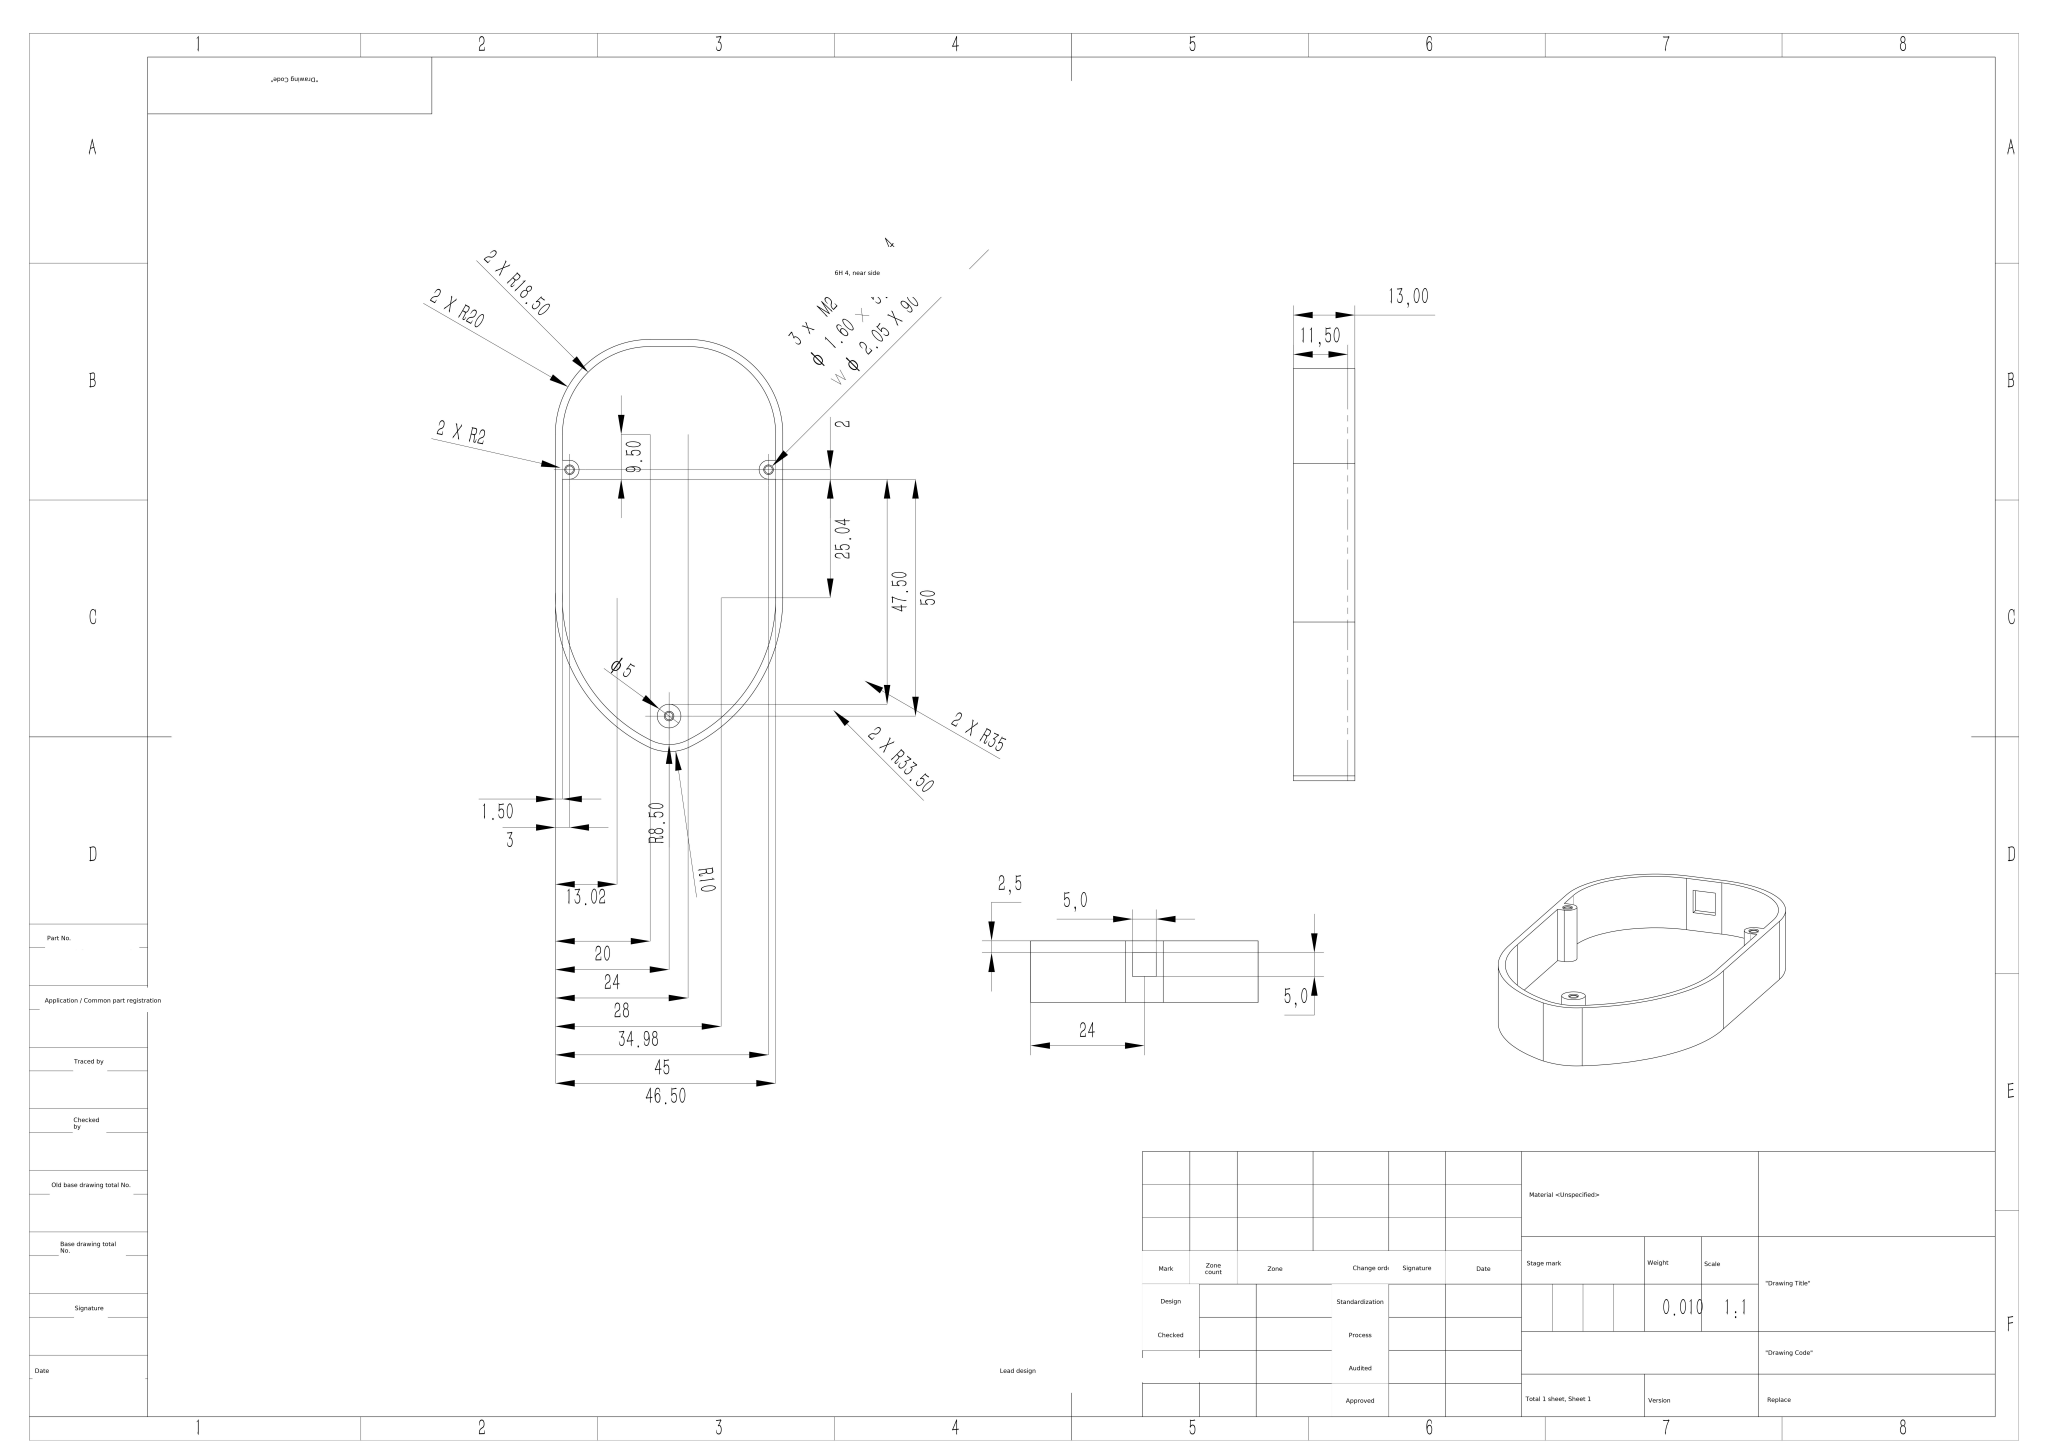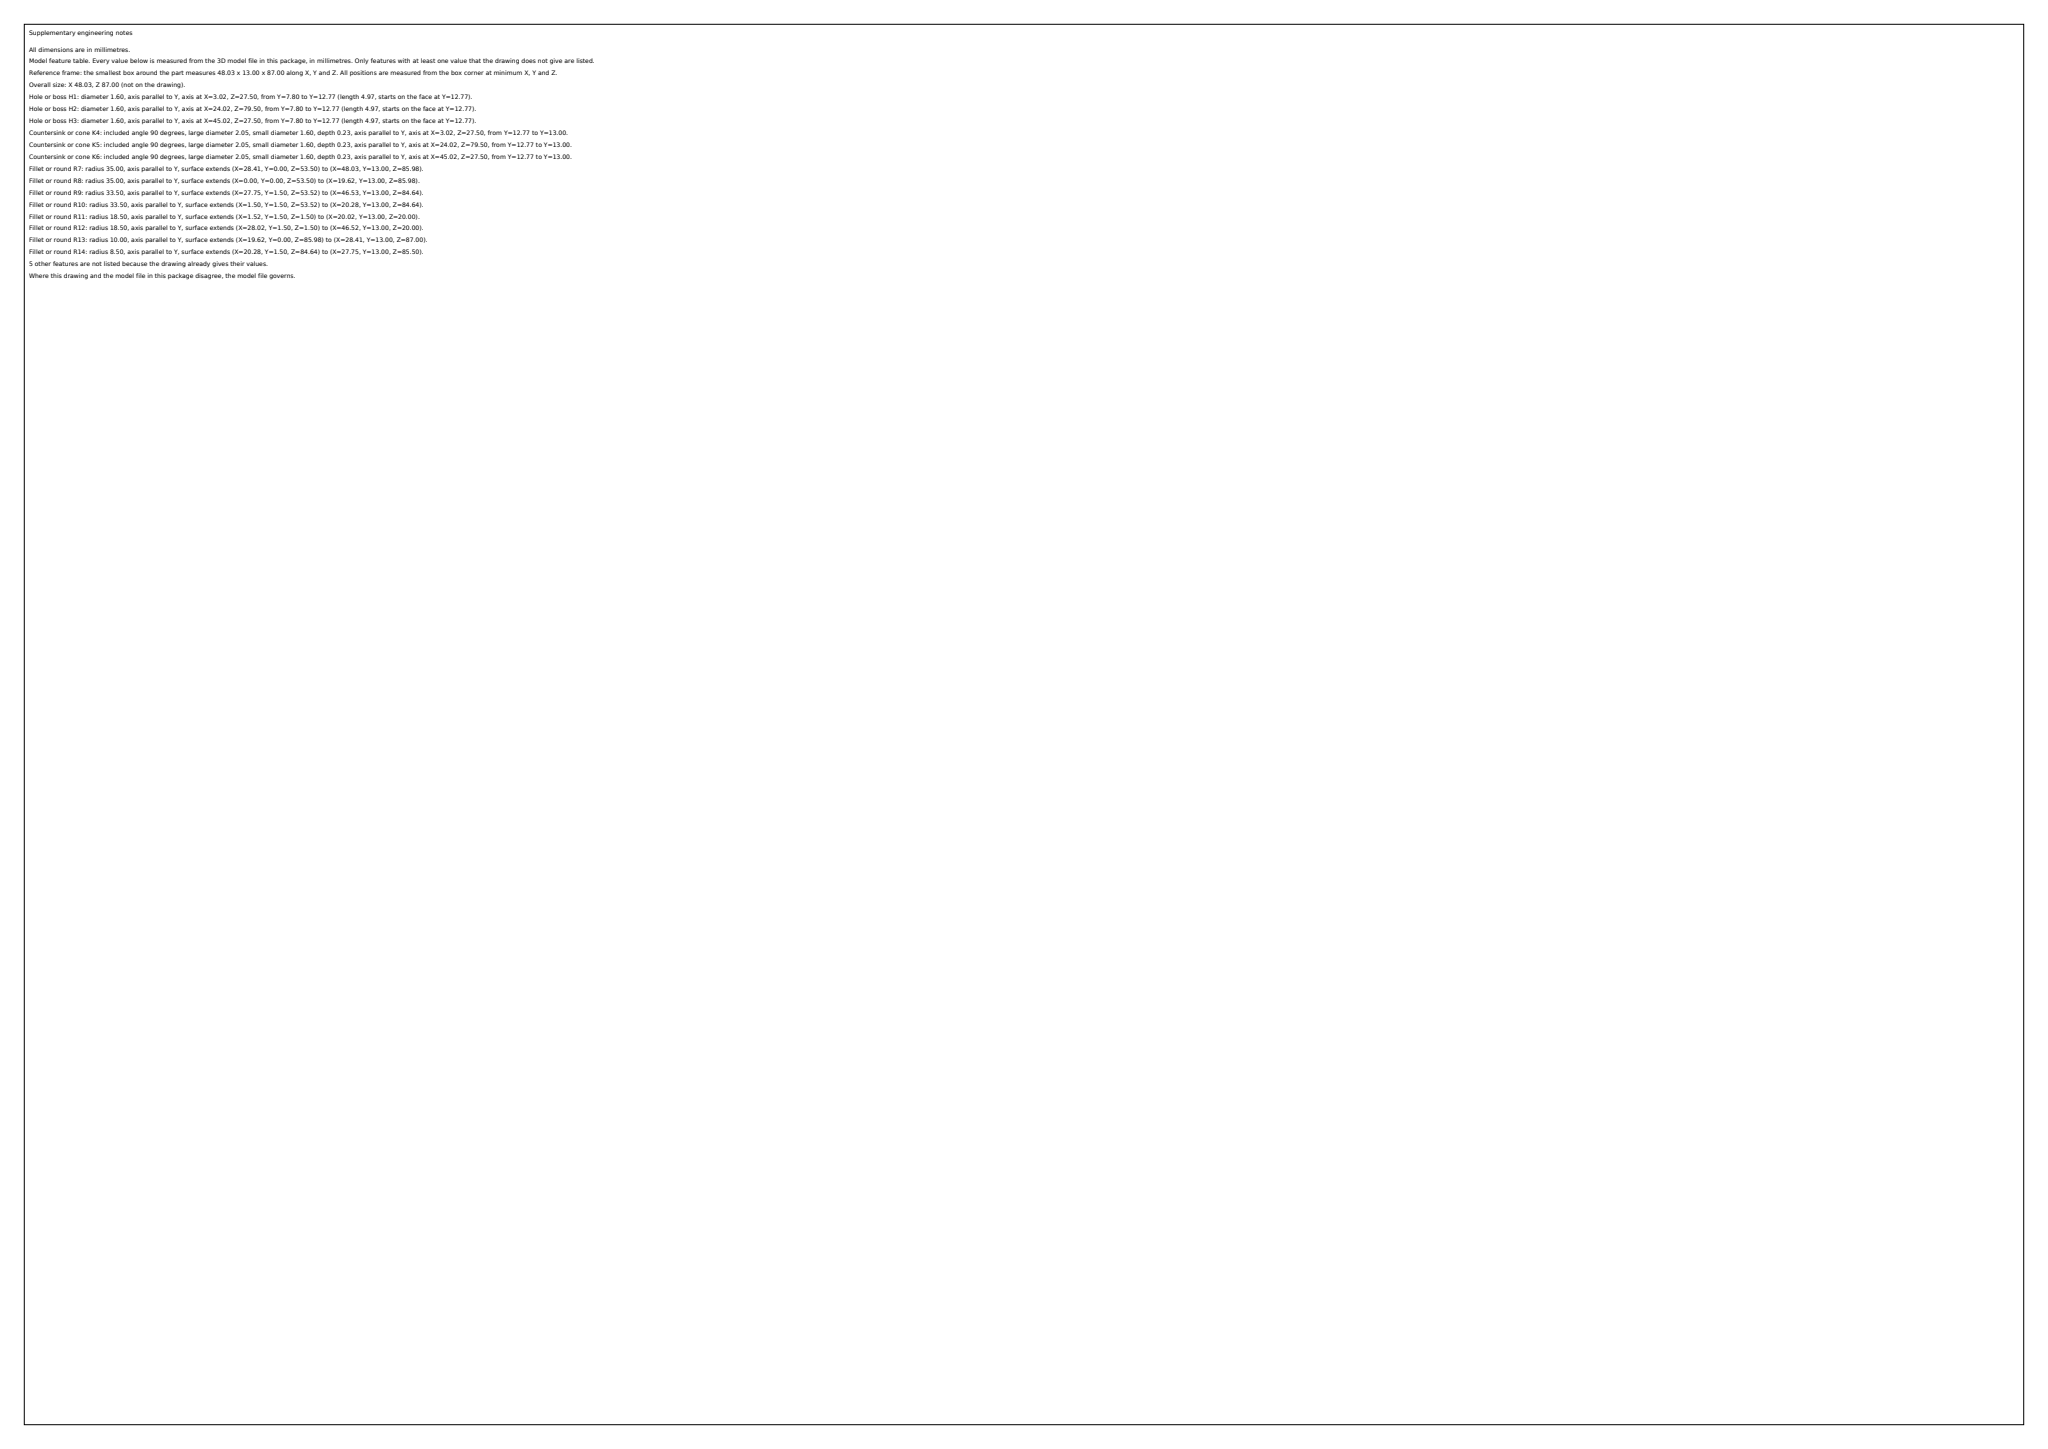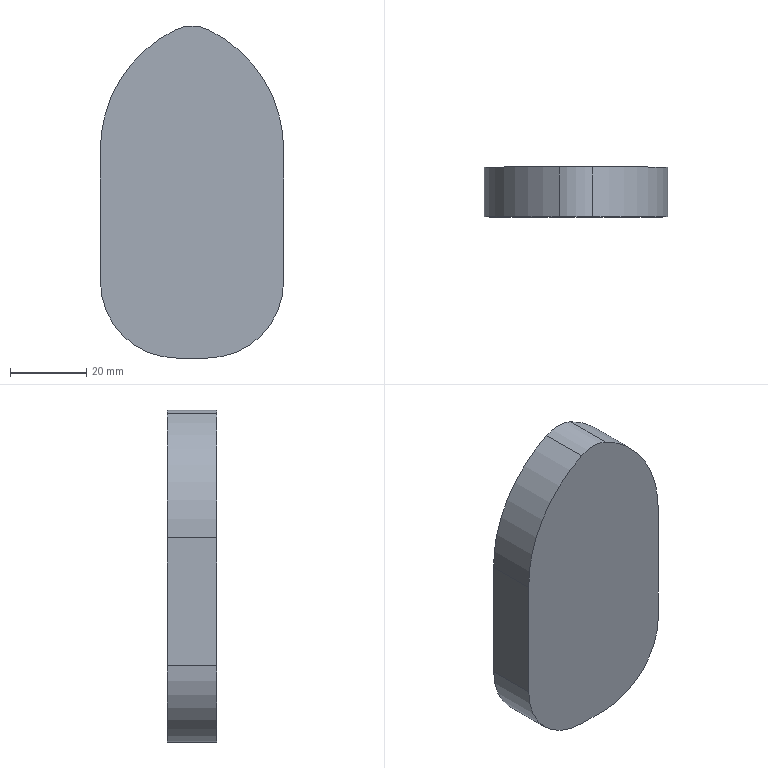Part | SolidWorks | mm | material <Unspecified> | 1 solid | 52 faces | box 48.03 x 13 x 87 mm | volume 9693 mm3 | cylinder 20 | plane 20 | cone 12 | commonest cylinder face diameters 1.6 x6 5 x2 70 x2 40 x2 67 x2 37 x2 4 x2 20 x1